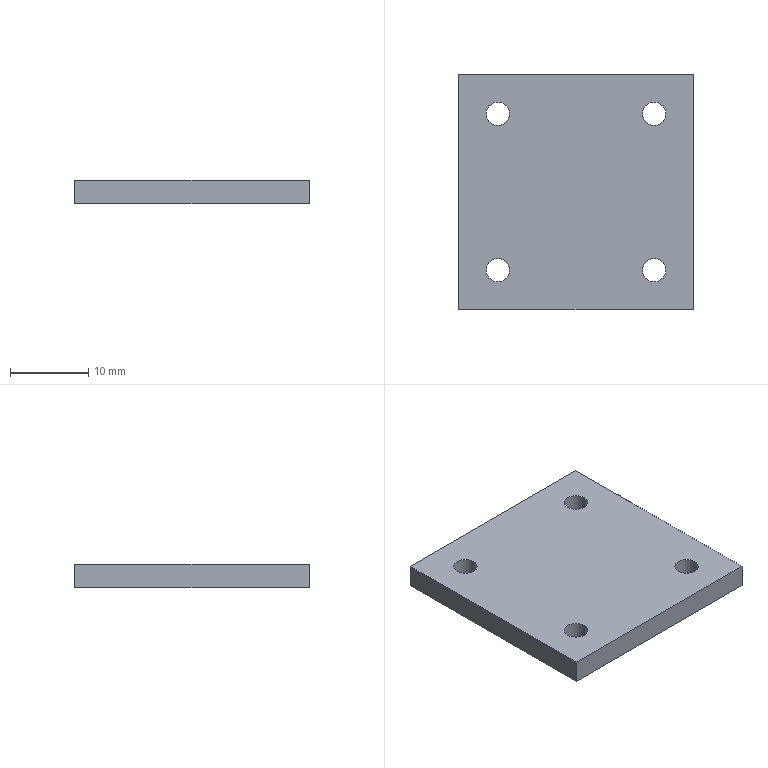Component | SolidWorks | Assembly3-1_Plate2-1 | 1 solid | 14 faces | box 30 x 30 x 3 mm | volume 2615 mm3 | cylinder 8 | plane 6 | commonest cylinder face diameters 3 x8
build123d program:
from build123d import *

# Parameters (mm, degrees)
SKETCH1_W           = 30
SKETCH1_H           = 30
SKETCH1_R           = 1.5
BOSS_EXTRUDE1_DEPTH = 3


with BuildPart() as part:
    # Sketch1 → Boss-Extrude1 (new body)
    with BuildSketch(Plane.XY):
        Rectangle(SKETCH1_W, SKETCH1_H)
        with Locations((-10, 10)):
            Circle(SKETCH1_R, mode=Mode.SUBTRACT)
        with Locations(Location((10, 10, 0), (0, 0, 180))):
            Circle(SKETCH1_R, mode=Mode.SUBTRACT)
        with Locations((10, -10)):
            Circle(SKETCH1_R, mode=Mode.SUBTRACT)
        with Locations(Location((-10, -10, 0), (0, 0, 180))):
            Circle(SKETCH1_R, mode=Mode.SUBTRACT)
    extrude(amount=BOSS_EXTRUDE1_DEPTH)


solid = part.part

# Placed as in the assembly
solid = solid.moved(Location((0, 35, 38), (0, 0, 0)))
STEP:
#1=COLOUR_RGB('',0.7922,0.8196,0.9333);
#2=FILL_AREA_STYLE_COLOUR('',#1);
#3=FILL_AREA_STYLE('',(#2));
#4=SURFACE_STYLE_FILL_AREA(#3);
#5=SURFACE_SIDE_STYLE('',(#4));
#6=SURFACE_STYLE_USAGE(.BOTH.,#5);
#7=PRESENTATION_STYLE_ASSIGNMENT((#6));
#8=CARTESIAN_POINT('',(-0.4528,1.772,1.496));
#9=VERTEX_POINT('',#8);
#10=CARTESIAN_POINT('',(-0.3346,1.772,1.496));
#11=VERTEX_POINT('',#10);
#12=CARTESIAN_POINT('',(-0.3937,1.772,1.496));
#13=DIRECTION('',(-0.,-0.,-1.));
#14=DIRECTION('',(-1.,0.,0.));
#15=AXIS2_PLACEMENT_3D('',#12,#13,#14);
#16=CIRCLE('',#15,0.05906);
#17=EDGE_CURVE('',#9,#11,#16,.T.);
#18=ORIENTED_EDGE('',*,*,#17,.T.);
#19=CARTESIAN_POINT('',(-0.3346,1.772,1.614));
#20=VERTEX_POINT('',#19);
#21=CARTESIAN_POINT('',(-0.3346,1.772,1.496));
#22=DIRECTION('',(0.,0.,1.));
#23=VECTOR('',#22,39.37);
#24=LINE('',#21,#23);
#25=EDGE_CURVE('',#11,#20,#24,.T.);
#26=ORIENTED_EDGE('',*,*,#25,.T.);
#27=CARTESIAN_POINT('',(-0.4528,1.772,1.614));
#28=VERTEX_POINT('',#27);
#29=CARTESIAN_POINT('',(-0.3937,1.772,1.614));
#30=DIRECTION('',(-0.,-0.,-1.));
#31=DIRECTION('',(-1.,0.,0.));
#32=AXIS2_PLACEMENT_3D('',#29,#30,#31);
#33=CIRCLE('',#32,0.05906);
#34=EDGE_CURVE('',#28,#20,#33,.T.);
#35=ORIENTED_EDGE('',*,*,#34,.F.);
#36=CARTESIAN_POINT('',(-0.4528,1.772,1.496));
#37=DIRECTION('',(0.,0.,1.));
#38=VECTOR('',#37,39.37);
#39=LINE('',#36,#38);
#40=EDGE_CURVE('',#9,#28,#39,.T.);
#41=ORIENTED_EDGE('',*,*,#40,.F.);
#42=EDGE_LOOP('',(#18,#26,#35,#41));
#43=FACE_OUTER_BOUND('',#42,.T.);
#44=CARTESIAN_POINT('',(-0.3937,1.772,1.496));
#45=DIRECTION('',(0.,0.,1.));
#46=DIRECTION('',(-1.,0.,0.));
#47=AXIS2_PLACEMENT_3D('',#44,#45,#46);
#48=CYLINDRICAL_SURFACE('',#47,0.05906);
#49=ADVANCED_FACE('',(#43),#48,.F.);
#50=CARTESIAN_POINT('',(0.3346,1.772,1.496));
#51=VERTEX_POINT('',#50);
#52=CARTESIAN_POINT('',(0.4528,1.772,1.496));
#53=VERTEX_POINT('',#52);
#54=CARTESIAN_POINT('',(0.3937,1.772,1.496));
#55=DIRECTION('',(-0.,-0.,-1.));
#56=DIRECTION('',(1.,0.,0.));
#57=AXIS2_PLACEMENT_3D('',#54,#55,#56);
#58=CIRCLE('',#57,0.05906);
#59=EDGE_CURVE('',#51,#53,#58,.T.);
#60=ORIENTED_EDGE('',*,*,#59,.T.);
#61=CARTESIAN_POINT('',(0.4528,1.772,1.614));
#62=VERTEX_POINT('',#61);
#63=CARTESIAN_POINT('',(0.4528,1.772,1.496));
#64=DIRECTION('',(0.,0.,1.));
#65=VECTOR('',#64,39.37);
#66=LINE('',#63,#65);
#67=EDGE_CURVE('',#53,#62,#66,.T.);
#68=ORIENTED_EDGE('',*,*,#67,.T.);
#69=CARTESIAN_POINT('',(0.3346,1.772,1.614));
#70=VERTEX_POINT('',#69);
#71=CARTESIAN_POINT('',(0.3937,1.772,1.614));
#72=DIRECTION('',(-0.,-0.,-1.));
#73=DIRECTION('',(1.,0.,0.));
#74=AXIS2_PLACEMENT_3D('',#71,#72,#73);
#75=CIRCLE('',#74,0.05906);
#76=EDGE_CURVE('',#70,#62,#75,.T.);
#77=ORIENTED_EDGE('',*,*,#76,.F.);
#78=CARTESIAN_POINT('',(0.3346,1.772,1.496));
#79=DIRECTION('',(0.,0.,1.));
#80=VECTOR('',#79,39.37);
#81=LINE('',#78,#80);
#82=EDGE_CURVE('',#51,#70,#81,.T.);
#83=ORIENTED_EDGE('',*,*,#82,.F.);
#84=EDGE_LOOP('',(#60,#68,#77,#83));
#85=FACE_OUTER_BOUND('',#84,.T.);
#86=CARTESIAN_POINT('',(0.3937,1.772,1.496));
#87=DIRECTION('',(0.,0.,1.));
#88=DIRECTION('',(-1.,0.,0.));
#89=AXIS2_PLACEMENT_3D('',#86,#87,#88);
#90=CYLINDRICAL_SURFACE('',#89,0.05906);
#91=ADVANCED_FACE('',(#85),#90,.F.);
#92=CARTESIAN_POINT('',(0.3346,0.9843,1.496));
#93=VERTEX_POINT('',#92);
#94=CARTESIAN_POINT('',(0.4528,0.9843,1.496));
#95=VERTEX_POINT('',#94);
#96=CARTESIAN_POINT('',(0.3937,0.9843,1.496));
#97=DIRECTION('',(-0.,-0.,-1.));
#98=DIRECTION('',(-1.,0.,0.));
#99=AXIS2_PLACEMENT_3D('',#96,#97,#98);
#100=CIRCLE('',#99,0.05906);
#101=EDGE_CURVE('',#93,#95,#100,.T.);
#102=ORIENTED_EDGE('',*,*,#101,.T.);
#103=CARTESIAN_POINT('',(0.4528,0.9843,1.614));
#104=VERTEX_POINT('',#103);
#105=CARTESIAN_POINT('',(0.4528,0.9843,1.496));
#106=DIRECTION('',(0.,0.,1.));
#107=VECTOR('',#106,39.37);
#108=LINE('',#105,#107);
#109=EDGE_CURVE('',#95,#104,#108,.T.);
#110=ORIENTED_EDGE('',*,*,#109,.T.);
#111=CARTESIAN_POINT('',(0.3346,0.9843,1.614));
#112=VERTEX_POINT('',#111);
#113=CARTESIAN_POINT('',(0.3937,0.9843,1.614));
#114=DIRECTION('',(-0.,-0.,-1.));
#115=DIRECTION('',(-1.,0.,0.));
#116=AXIS2_PLACEMENT_3D('',#113,#114,#115);
#117=CIRCLE('',#116,0.05906);
#118=EDGE_CURVE('',#112,#104,#117,.T.);
#119=ORIENTED_EDGE('',*,*,#118,.F.);
#120=CARTESIAN_POINT('',(0.3346,0.9843,1.496));
#121=DIRECTION('',(0.,0.,1.));
#122=VECTOR('',#121,39.37);
#123=LINE('',#120,#122);
#124=EDGE_CURVE('',#93,#112,#123,.T.);
#125=ORIENTED_EDGE('',*,*,#124,.F.);
#126=EDGE_LOOP('',(#102,#110,#119,#125));
#127=FACE_OUTER_BOUND('',#126,.T.);
#128=CARTESIAN_POINT('',(0.3937,0.9843,1.496));
#129=DIRECTION('',(0.,0.,1.));
#130=DIRECTION('',(-1.,0.,0.));
#131=AXIS2_PLACEMENT_3D('',#128,#129,#130);
#132=CYLINDRICAL_SURFACE('',#131,0.05906);
#133=ADVANCED_FACE('',(#127),#132,.F.);
#134=CARTESIAN_POINT('',(-0.4528,0.9843,1.496));
#135=VERTEX_POINT('',#134);
#136=CARTESIAN_POINT('',(-0.3346,0.9843,1.496));
#137=VERTEX_POINT('',#136);
#138=CARTESIAN_POINT('',(-0.3937,0.9843,1.496));
#139=DIRECTION('',(-0.,-0.,-1.));
#140=DIRECTION('',(1.,0.,0.));
#141=AXIS2_PLACEMENT_3D('',#138,#139,#140);
#142=CIRCLE('',#141,0.05906);
#143=EDGE_CURVE('',#135,#137,#142,.T.);
#144=ORIENTED_EDGE('',*,*,#143,.T.);
#145=CARTESIAN_POINT('',(-0.3346,0.9843,1.614));
#146=VERTEX_POINT('',#145);
#147=CARTESIAN_POINT('',(-0.3346,0.9843,1.496));
#148=DIRECTION('',(0.,0.,1.));
#149=VECTOR('',#148,39.37);
#150=LINE('',#147,#149);
#151=EDGE_CURVE('',#137,#146,#150,.T.);
#152=ORIENTED_EDGE('',*,*,#151,.T.);
#153=CARTESIAN_POINT('',(-0.4528,0.9843,1.614));
#154=VERTEX_POINT('',#153);
#155=CARTESIAN_POINT('',(-0.3937,0.9843,1.614));
#156=DIRECTION('',(-0.,-0.,-1.));
#157=DIRECTION('',(1.,0.,0.));
#158=AXIS2_PLACEMENT_3D('',#155,#156,#157);
#159=CIRCLE('',#158,0.05906);
#160=EDGE_CURVE('',#154,#146,#159,.T.);
#161=ORIENTED_EDGE('',*,*,#160,.F.);
#162=CARTESIAN_POINT('',(-0.4528,0.9843,1.496));
#163=DIRECTION('',(0.,0.,1.));
#164=VECTOR('',#163,39.37);
#165=LINE('',#162,#164);
#166=EDGE_CURVE('',#135,#154,#165,.T.);
#167=ORIENTED_EDGE('',*,*,#166,.F.);
#168=EDGE_LOOP('',(#144,#152,#161,#167));
#169=FACE_OUTER_BOUND('',#168,.T.);
#170=CARTESIAN_POINT('',(-0.3937,0.9843,1.496));
#171=DIRECTION('',(0.,0.,1.));
#172=DIRECTION('',(-1.,0.,0.));
#173=AXIS2_PLACEMENT_3D('',#170,#171,#172);
#174=CYLINDRICAL_SURFACE('',#173,0.05906);
#175=ADVANCED_FACE('',(#169),#174,.F.);
#176=CARTESIAN_POINT('',(0.5906,1.969,1.496));
#177=VERTEX_POINT('',#176);
#178=CARTESIAN_POINT('',(0.5906,0.7874,1.496));
#179=VERTEX_POINT('',#178);
#180=CARTESIAN_POINT('',(0.5906,1.969,1.496));
#181=DIRECTION('',(0.,-1.,0.));
#182=VECTOR('',#181,39.37);
#183=LINE('',#180,#182);
#184=EDGE_CURVE('',#177,#179,#183,.T.);
#185=ORIENTED_EDGE('',*,*,#184,.T.);
#186=CARTESIAN_POINT('',(-0.5906,0.7874,1.496));
#187=VERTEX_POINT('',#186);
#188=CARTESIAN_POINT('',(-0.5906,0.7874,1.496));
#189=DIRECTION('',(-1.,-0.,0.));
#190=VECTOR('',#189,39.37);
#191=LINE('',#188,#190);
#192=EDGE_CURVE('',#179,#187,#191,.T.);
#193=ORIENTED_EDGE('',*,*,#192,.T.);
#194=CARTESIAN_POINT('',(-0.5906,1.969,1.496));
#195=VERTEX_POINT('',#194);
#196=CARTESIAN_POINT('',(-0.5906,1.969,1.496));
#197=DIRECTION('',(-0.,1.,-0.));
#198=VECTOR('',#197,39.37);
#199=LINE('',#196,#198);
#200=EDGE_CURVE('',#187,#195,#199,.T.);
#201=ORIENTED_EDGE('',*,*,#200,.T.);
#202=CARTESIAN_POINT('',(-0.5906,1.969,1.496));
#203=DIRECTION('',(1.,0.,-0.));
#204=VECTOR('',#203,39.37);
#205=LINE('',#202,#204);
#206=EDGE_CURVE('',#195,#177,#205,.T.);
#207=ORIENTED_EDGE('',*,*,#206,.T.);
#208=EDGE_LOOP('',(#185,#193,#201,#207));
#209=FACE_OUTER_BOUND('',#208,.T.);
#210=ORIENTED_EDGE('',*,*,#143,.F.);
#211=CARTESIAN_POINT('',(-0.3937,0.9843,1.496));
#212=DIRECTION('',(-0.,-0.,-1.));
#213=DIRECTION('',(1.,0.,0.));
#214=AXIS2_PLACEMENT_3D('',#211,#212,#213);
#215=CIRCLE('',#214,0.05906);
#216=EDGE_CURVE('',#137,#135,#215,.T.);
#217=ORIENTED_EDGE('',*,*,#216,.F.);
#218=EDGE_LOOP('',(#210,#217));
#219=FACE_BOUND('',#218,.T.);
#220=ORIENTED_EDGE('',*,*,#101,.F.);
#221=CARTESIAN_POINT('',(0.3937,0.9843,1.496));
#222=DIRECTION('',(-0.,-0.,-1.));
#223=DIRECTION('',(-1.,0.,0.));
#224=AXIS2_PLACEMENT_3D('',#221,#222,#223);
#225=CIRCLE('',#224,0.05906);
#226=EDGE_CURVE('',#95,#93,#225,.T.);
#227=ORIENTED_EDGE('',*,*,#226,.F.);
#228=EDGE_LOOP('',(#220,#227));
#229=FACE_BOUND('',#228,.T.);
#230=ORIENTED_EDGE('',*,*,#59,.F.);
#231=CARTESIAN_POINT('',(0.3937,1.772,1.496));
#232=DIRECTION('',(-0.,-0.,-1.));
#233=DIRECTION('',(1.,0.,0.));
#234=AXIS2_PLACEMENT_3D('',#231,#232,#233);
#235=CIRCLE('',#234,0.05906);
#236=EDGE_CURVE('',#53,#51,#235,.T.);
#237=ORIENTED_EDGE('',*,*,#236,.F.);
#238=EDGE_LOOP('',(#230,#237));
#239=FACE_BOUND('',#238,.T.);
#240=ORIENTED_EDGE('',*,*,#17,.F.);
#241=CARTESIAN_POINT('',(-0.3937,1.772,1.496));
#242=DIRECTION('',(-0.,-0.,-1.));
#243=DIRECTION('',(-1.,0.,0.));
#244=AXIS2_PLACEMENT_3D('',#241,#242,#243);
#245=CIRCLE('',#244,0.05906);
#246=EDGE_CURVE('',#11,#9,#245,.T.);
#247=ORIENTED_EDGE('',*,*,#246,.F.);
#248=EDGE_LOOP('',(#240,#247));
#249=FACE_BOUND('',#248,.T.);
#250=CARTESIAN_POINT('',(0.,1.378,1.496));
#251=DIRECTION('',(0.,0.,1.));
#252=DIRECTION('',(-1.,-0.,0.));
#253=AXIS2_PLACEMENT_3D('',#250,#251,#252);
#254=PLANE('',#253);
#255=ADVANCED_FACE('',(#209,#219,#229,#239,#249),#254,.F.);
#256=ORIENTED_EDGE('',*,*,#76,.T.);
#257=CARTESIAN_POINT('',(0.3937,1.772,1.614));
#258=DIRECTION('',(-0.,-0.,-1.));
#259=DIRECTION('',(1.,0.,0.));
#260=AXIS2_PLACEMENT_3D('',#257,#258,#259);
#261=CIRCLE('',#260,0.05906);
#262=EDGE_CURVE('',#62,#70,#261,.T.);
#263=ORIENTED_EDGE('',*,*,#262,.T.);
#264=EDGE_LOOP('',(#256,#263));
#265=FACE_BOUND('',#264,.T.);
#266=ORIENTED_EDGE('',*,*,#160,.T.);
#267=CARTESIAN_POINT('',(-0.3937,0.9843,1.614));
#268=DIRECTION('',(-0.,-0.,-1.));
#269=DIRECTION('',(1.,0.,0.));
#270=AXIS2_PLACEMENT_3D('',#267,#268,#269);
#271=CIRCLE('',#270,0.05906);
#272=EDGE_CURVE('',#146,#154,#271,.T.);
#273=ORIENTED_EDGE('',*,*,#272,.T.);
#274=EDGE_LOOP('',(#266,#273));
#275=FACE_BOUND('',#274,.T.);
#276=CARTESIAN_POINT('',(0.5906,1.969,1.614));
#277=VERTEX_POINT('',#276);
#278=CARTESIAN_POINT('',(0.5906,0.7874,1.614));
#279=VERTEX_POINT('',#278);
#280=CARTESIAN_POINT('',(0.5906,1.969,1.614));
#281=DIRECTION('',(0.,-1.,0.));
#282=VECTOR('',#281,39.37);
#283=LINE('',#280,#282);
#284=EDGE_CURVE('',#277,#279,#283,.T.);
#285=ORIENTED_EDGE('',*,*,#284,.F.);
#286=CARTESIAN_POINT('',(-0.5906,1.969,1.614));
#287=VERTEX_POINT('',#286);
#288=CARTESIAN_POINT('',(-0.5906,1.969,1.614));
#289=DIRECTION('',(1.,0.,-0.));
#290=VECTOR('',#289,39.37);
#291=LINE('',#288,#290);
#292=EDGE_CURVE('',#287,#277,#291,.T.);
#293=ORIENTED_EDGE('',*,*,#292,.F.);
#294=CARTESIAN_POINT('',(-0.5906,0.7874,1.614));
#295=VERTEX_POINT('',#294);
#296=CARTESIAN_POINT('',(-0.5906,1.969,1.614));
#297=DIRECTION('',(-0.,1.,-0.));
#298=VECTOR('',#297,39.37);
#299=LINE('',#296,#298);
#300=EDGE_CURVE('',#295,#287,#299,.T.);
#301=ORIENTED_EDGE('',*,*,#300,.F.);
#302=CARTESIAN_POINT('',(-0.5906,0.7874,1.614));
#303=DIRECTION('',(-1.,-0.,0.));
#304=VECTOR('',#303,39.37);
#305=LINE('',#302,#304);
#306=EDGE_CURVE('',#279,#295,#305,.T.);
#307=ORIENTED_EDGE('',*,*,#306,.F.);
#308=EDGE_LOOP('',(#285,#293,#301,#307));
#309=FACE_OUTER_BOUND('',#308,.T.);
#310=ORIENTED_EDGE('',*,*,#118,.T.);
#311=CARTESIAN_POINT('',(0.3937,0.9843,1.614));
#312=DIRECTION('',(-0.,-0.,-1.));
#313=DIRECTION('',(-1.,0.,0.));
#314=AXIS2_PLACEMENT_3D('',#311,#312,#313);
#315=CIRCLE('',#314,0.05906);
#316=EDGE_CURVE('',#104,#112,#315,.T.);
#317=ORIENTED_EDGE('',*,*,#316,.T.);
#318=EDGE_LOOP('',(#310,#317));
#319=FACE_BOUND('',#318,.T.);
#320=ORIENTED_EDGE('',*,*,#34,.T.);
#321=CARTESIAN_POINT('',(-0.3937,1.772,1.614));
#322=DIRECTION('',(-0.,-0.,-1.));
#323=DIRECTION('',(-1.,0.,0.));
#324=AXIS2_PLACEMENT_3D('',#321,#322,#323);
#325=CIRCLE('',#324,0.05906);
#326=EDGE_CURVE('',#20,#28,#325,.T.);
#327=ORIENTED_EDGE('',*,*,#326,.T.);
#328=EDGE_LOOP('',(#320,#327));
#329=FACE_BOUND('',#328,.T.);
#330=CARTESIAN_POINT('',(0.,1.378,1.614));
#331=DIRECTION('',(0.,0.,1.));
#332=DIRECTION('',(-1.,-0.,0.));
#333=AXIS2_PLACEMENT_3D('',#330,#331,#332);
#334=PLANE('',#333);
#335=ADVANCED_FACE('',(#265,#275,#309,#319,#329),#334,.T.);
#336=ORIENTED_EDGE('',*,*,#284,.T.);
#337=CARTESIAN_POINT('',(0.5906,0.7874,1.496));
#338=DIRECTION('',(0.,0.,1.));
#339=VECTOR('',#338,39.37);
#340=LINE('',#337,#339);
#341=EDGE_CURVE('',#179,#279,#340,.T.);
#342=ORIENTED_EDGE('',*,*,#341,.F.);
#343=ORIENTED_EDGE('',*,*,#184,.F.);
#344=CARTESIAN_POINT('',(0.5906,1.969,1.496));
#345=DIRECTION('',(0.,0.,1.));
#346=VECTOR('',#345,39.37);
#347=LINE('',#344,#346);
#348=EDGE_CURVE('',#177,#277,#347,.T.);
#349=ORIENTED_EDGE('',*,*,#348,.T.);
#350=EDGE_LOOP('',(#336,#342,#343,#349));
#351=FACE_OUTER_BOUND('',#350,.T.);
#352=CARTESIAN_POINT('',(0.5906,1.969,1.496));
#353=DIRECTION('',(-1.,-0.,0.));
#354=DIRECTION('',(-0.,-0.,-1.));
#355=AXIS2_PLACEMENT_3D('',#352,#353,#354);
#356=PLANE('',#355);
#357=ADVANCED_FACE('',(#351),#356,.F.);
#358=ORIENTED_EDGE('',*,*,#306,.T.);
#359=CARTESIAN_POINT('',(-0.5906,0.7874,1.496));
#360=DIRECTION('',(0.,0.,1.));
#361=VECTOR('',#360,39.37);
#362=LINE('',#359,#361);
#363=EDGE_CURVE('',#187,#295,#362,.T.);
#364=ORIENTED_EDGE('',*,*,#363,.F.);
#365=ORIENTED_EDGE('',*,*,#192,.F.);
#366=ORIENTED_EDGE('',*,*,#341,.T.);
#367=EDGE_LOOP('',(#358,#364,#365,#366));
#368=FACE_OUTER_BOUND('',#367,.T.);
#369=CARTESIAN_POINT('',(-0.5906,0.7874,1.496));
#370=DIRECTION('',(-0.,1.,-0.));
#371=DIRECTION('',(0.,0.,1.));
#372=AXIS2_PLACEMENT_3D('',#369,#370,#371);
#373=PLANE('',#372);
#374=ADVANCED_FACE('',(#368),#373,.F.);
#375=ORIENTED_EDGE('',*,*,#300,.T.);
#376=CARTESIAN_POINT('',(-0.5906,1.969,1.496));
#377=DIRECTION('',(0.,0.,1.));
#378=VECTOR('',#377,39.37);
#379=LINE('',#376,#378);
#380=EDGE_CURVE('',#195,#287,#379,.T.);
#381=ORIENTED_EDGE('',*,*,#380,.F.);
#382=ORIENTED_EDGE('',*,*,#200,.F.);
#383=ORIENTED_EDGE('',*,*,#363,.T.);
#384=EDGE_LOOP('',(#375,#381,#382,#383));
#385=FACE_OUTER_BOUND('',#384,.T.);
#386=CARTESIAN_POINT('',(-0.5906,1.969,1.496));
#387=DIRECTION('',(1.,0.,-0.));
#388=DIRECTION('',(0.,0.,1.));
#389=AXIS2_PLACEMENT_3D('',#386,#387,#388);
#390=PLANE('',#389);
#391=ADVANCED_FACE('',(#385),#390,.F.);
#392=ORIENTED_EDGE('',*,*,#292,.T.);
#393=ORIENTED_EDGE('',*,*,#348,.F.);
#394=ORIENTED_EDGE('',*,*,#206,.F.);
#395=ORIENTED_EDGE('',*,*,#380,.T.);
#396=EDGE_LOOP('',(#392,#393,#394,#395));
#397=FACE_OUTER_BOUND('',#396,.T.);
#398=CARTESIAN_POINT('',(-0.5906,1.969,1.496));
#399=DIRECTION('',(0.,-1.,0.));
#400=DIRECTION('',(-0.,-0.,-1.));
#401=AXIS2_PLACEMENT_3D('',#398,#399,#400);
#402=PLANE('',#401);
#403=ADVANCED_FACE('',(#397),#402,.F.);
#404=ORIENTED_EDGE('',*,*,#151,.F.);
#405=ORIENTED_EDGE('',*,*,#216,.T.);
#406=ORIENTED_EDGE('',*,*,#166,.T.);
#407=ORIENTED_EDGE('',*,*,#272,.F.);
#408=EDGE_LOOP('',(#404,#405,#406,#407));
#409=FACE_OUTER_BOUND('',#408,.T.);
#410=CARTESIAN_POINT('',(-0.3937,0.9843,1.496));
#411=DIRECTION('',(0.,0.,1.));
#412=DIRECTION('',(-1.,0.,0.));
#413=AXIS2_PLACEMENT_3D('',#410,#411,#412);
#414=CYLINDRICAL_SURFACE('',#413,0.05906);
#415=ADVANCED_FACE('',(#409),#414,.F.);
#416=ORIENTED_EDGE('',*,*,#109,.F.);
#417=ORIENTED_EDGE('',*,*,#226,.T.);
#418=ORIENTED_EDGE('',*,*,#124,.T.);
#419=ORIENTED_EDGE('',*,*,#316,.F.);
#420=EDGE_LOOP('',(#416,#417,#418,#419));
#421=FACE_OUTER_BOUND('',#420,.T.);
#422=CARTESIAN_POINT('',(0.3937,0.9843,1.496));
#423=DIRECTION('',(0.,0.,1.));
#424=DIRECTION('',(-1.,0.,0.));
#425=AXIS2_PLACEMENT_3D('',#422,#423,#424);
#426=CYLINDRICAL_SURFACE('',#425,0.05906);
#427=ADVANCED_FACE('',(#421),#426,.F.);
#428=ORIENTED_EDGE('',*,*,#67,.F.);
#429=ORIENTED_EDGE('',*,*,#236,.T.);
#430=ORIENTED_EDGE('',*,*,#82,.T.);
#431=ORIENTED_EDGE('',*,*,#262,.F.);
#432=EDGE_LOOP('',(#428,#429,#430,#431));
#433=FACE_OUTER_BOUND('',#432,.T.);
#434=CARTESIAN_POINT('',(0.3937,1.772,1.496));
#435=DIRECTION('',(0.,0.,1.));
#436=DIRECTION('',(-1.,0.,0.));
#437=AXIS2_PLACEMENT_3D('',#434,#435,#436);
#438=CYLINDRICAL_SURFACE('',#437,0.05906);
#439=ADVANCED_FACE('',(#433),#438,.F.);
#440=ORIENTED_EDGE('',*,*,#25,.F.);
#441=ORIENTED_EDGE('',*,*,#246,.T.);
#442=ORIENTED_EDGE('',*,*,#40,.T.);
#443=ORIENTED_EDGE('',*,*,#326,.F.);
#444=EDGE_LOOP('',(#440,#441,#442,#443));
#445=FACE_OUTER_BOUND('',#444,.T.);
#446=CARTESIAN_POINT('',(-0.3937,1.772,1.496));
#447=DIRECTION('',(0.,0.,1.));
#448=DIRECTION('',(-1.,0.,0.));
#449=AXIS2_PLACEMENT_3D('',#446,#447,#448);
#450=CYLINDRICAL_SURFACE('',#449,0.05906);
#451=ADVANCED_FACE('',(#445),#450,.F.);
#452=CLOSED_SHELL('',(#49,#91,#133,#175,#255,#335,#357,#374,#391,#403,#415,#427,#439,#451));
#453=MANIFOLD_SOLID_BREP('',#452);
#454=STYLED_ITEM('',(#7),#453);
#455=(LENGTH_UNIT()NAMED_UNIT(*)SI_UNIT($,.METRE.));
#456=LENGTH_MEASURE_WITH_UNIT(LENGTH_MEASURE(0.0254),#455);
#457=DIMENSIONAL_EXPONENTS(1.,0.,0.,0.,0.,0.,0.);
#458=(CONVERSION_BASED_UNIT('',#456)LENGTH_UNIT()NAMED_UNIT(#457));
#459=UNCERTAINTY_MEASURE_WITH_UNIT(LENGTH_MEASURE(0.00001),#458,'','');
#460=(NAMED_UNIT(*)PLANE_ANGLE_UNIT()SI_UNIT($,.RADIAN.));
#461=(NAMED_UNIT(*)SI_UNIT($,.STERADIAN.)SOLID_ANGLE_UNIT());
#462=(GEOMETRIC_REPRESENTATION_CONTEXT(3)GLOBAL_UNCERTAINTY_ASSIGNED_CONTEXT((#459))GLOBAL_UNIT_ASSIGNED_CONTEXT((#458,#460,#461))REPRESENTATION_CONTEXT('',''));
#463=MECHANICAL_DESIGN_GEOMETRIC_PRESENTATION_REPRESENTATION('',(#454),#462);
#464=CARTESIAN_POINT('',(0.,0.,0.));
#465=DIRECTION('',(0.,0.,1.));
#466=DIRECTION('',(1.,0.,0.));
#467=AXIS2_PLACEMENT_3D('',#464,#465,#466);
#468=(LENGTH_UNIT()NAMED_UNIT(*)SI_UNIT($,.METRE.));
#469=LENGTH_MEASURE_WITH_UNIT(LENGTH_MEASURE(0.0254),#468);
#470=DIMENSIONAL_EXPONENTS(1.,0.,0.,0.,0.,0.,0.);
#471=(CONVERSION_BASED_UNIT('',#469)LENGTH_UNIT()NAMED_UNIT(#470));
#472=UNCERTAINTY_MEASURE_WITH_UNIT(LENGTH_MEASURE(0.00001),#471,'','');
#473=(NAMED_UNIT(*)PLANE_ANGLE_UNIT()SI_UNIT($,.RADIAN.));
#474=(NAMED_UNIT(*)SI_UNIT($,.STERADIAN.)SOLID_ANGLE_UNIT());
#475=(GEOMETRIC_REPRESENTATION_CONTEXT(3)GLOBAL_UNCERTAINTY_ASSIGNED_CONTEXT((#472))GLOBAL_UNIT_ASSIGNED_CONTEXT((#471,#473,#474))REPRESENTATION_CONTEXT('',''));
#476=ADVANCED_BREP_SHAPE_REPRESENTATION('',(#453,#467),#475);
#477=PRESENTATION_LAYER_ASSIGNMENT('','',(#454));